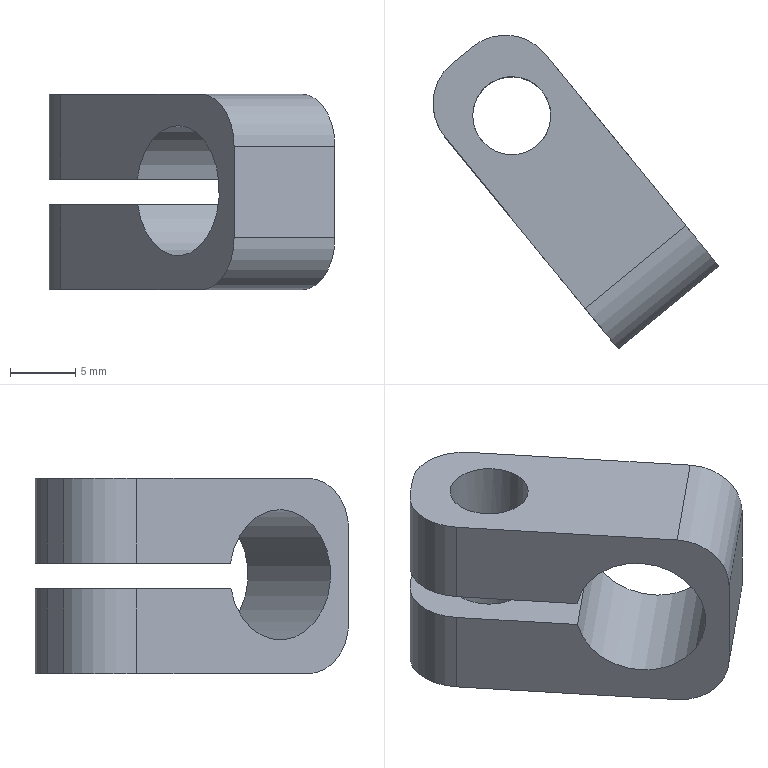Component | NX | BLOCK_1_2 | 1 solid | 18 faces | volume 2178 mm3 | plane 9 | cylinder 9 | commonest cylinder face diameters 8 x6 6 x2 10 x1